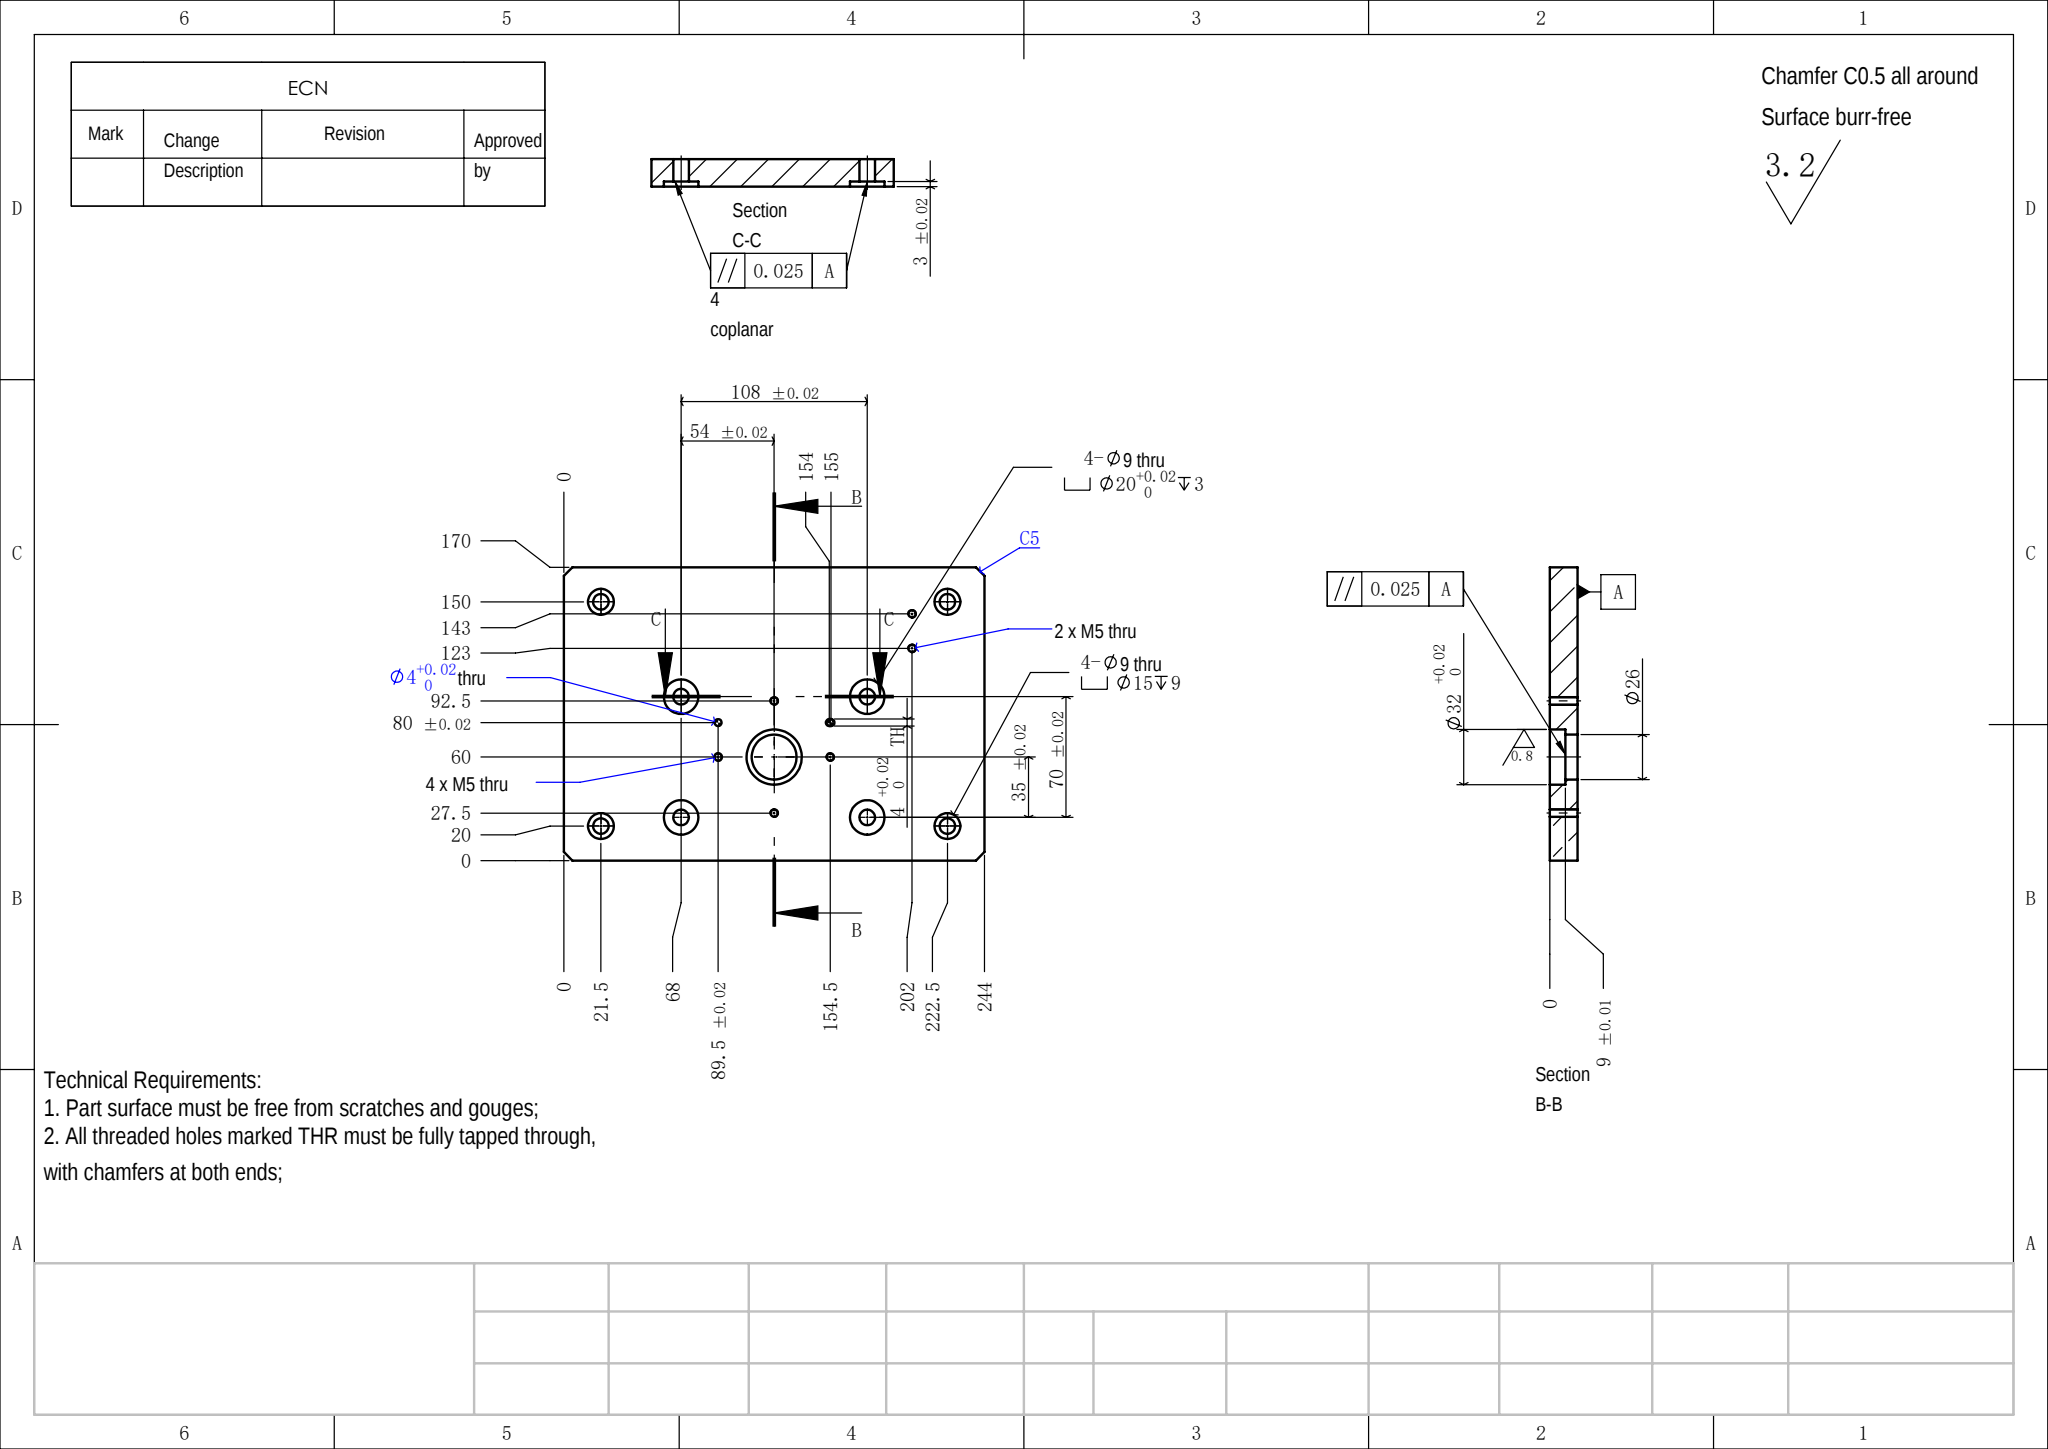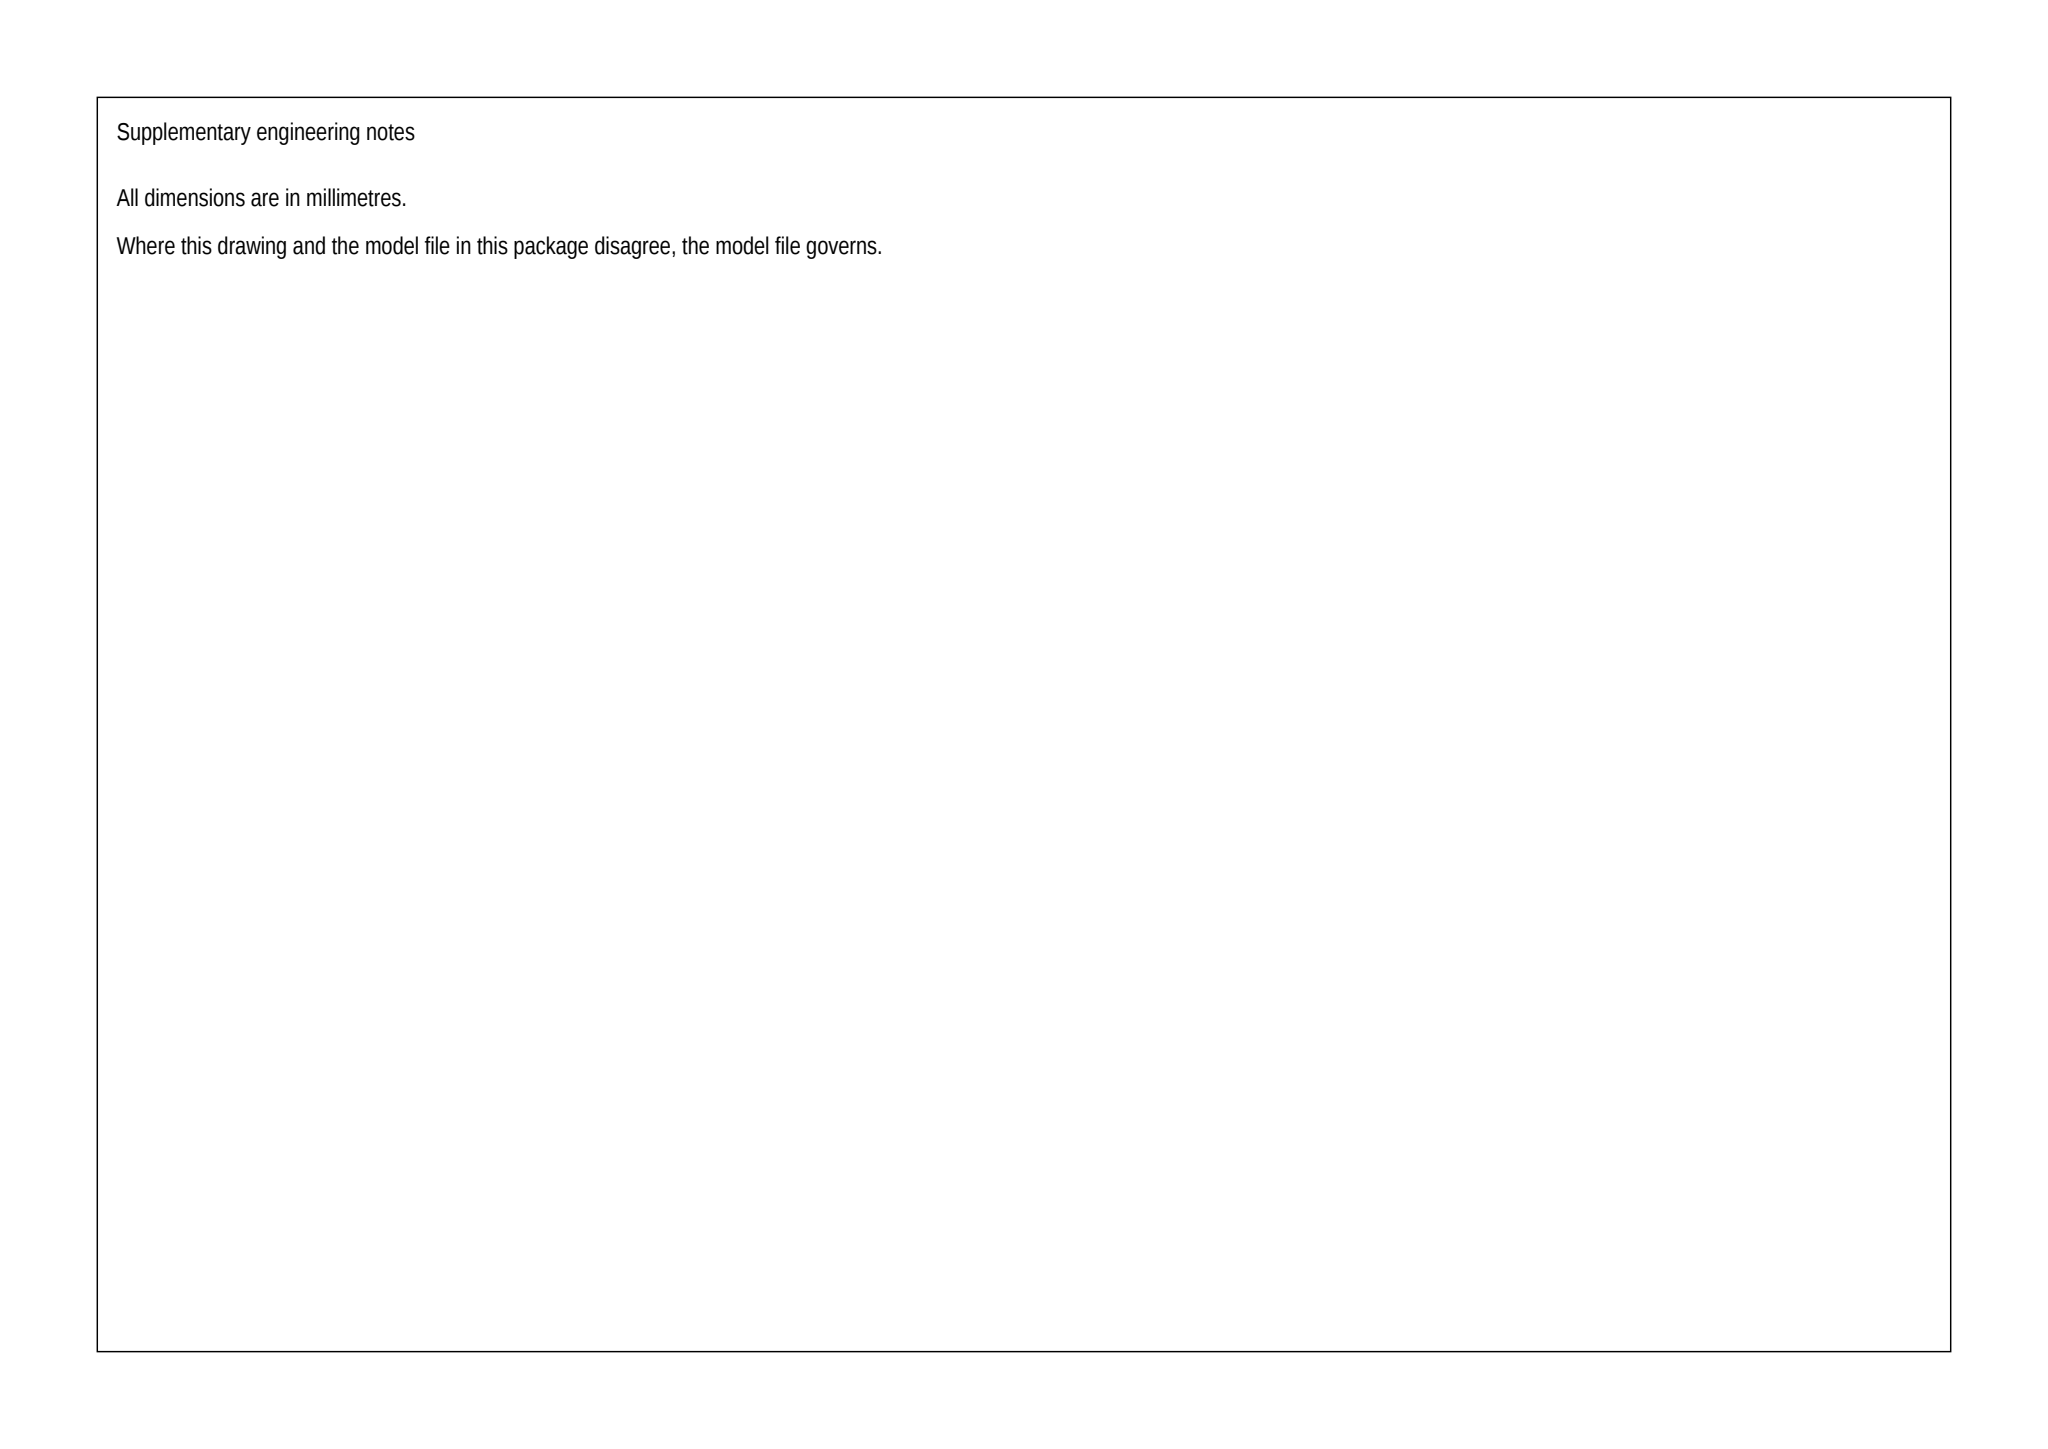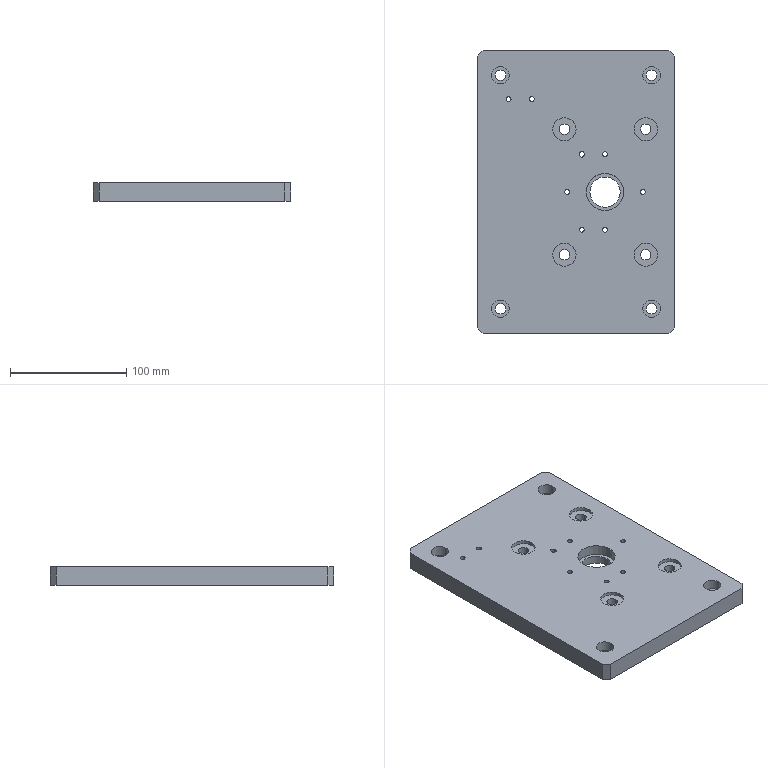Part | SolidWorks | mm | 1 solid | 73 faces | box 170 x 244 x 16 mm | volume 634908 mm3 | cylinder 52 | plane 21 | commonest cylinder face diameters 9 x16 4.2 x12 20 x8 15 x8 4 x4 26 x2 32 x2
Drawing notes:
OVERALL PLATE 170 x 244 x 16 THK | from the solid: bbox_xyz = [170,244,16]; z-planes at 0.0 and 16.0
4-Ø9 THRU, CBORE Ø15 DP 9 FROM OPP FACE | from the solid: Ø9 z-cyl len 7 at (20,21.5),(20,222.5),(150,21.5),(150,222.5); Ø15 same axes len 9 (7+9=16 THRU)
SECT 9B-B BORE: Ø26 DP 7 FROM A, Ø32 DP 9 OPP FACE, THRU | from the solid: Ø26 z-cyl len 7 and Ø32 z-cyl len 9 both at (110,122); 7+9=16 = plate thk